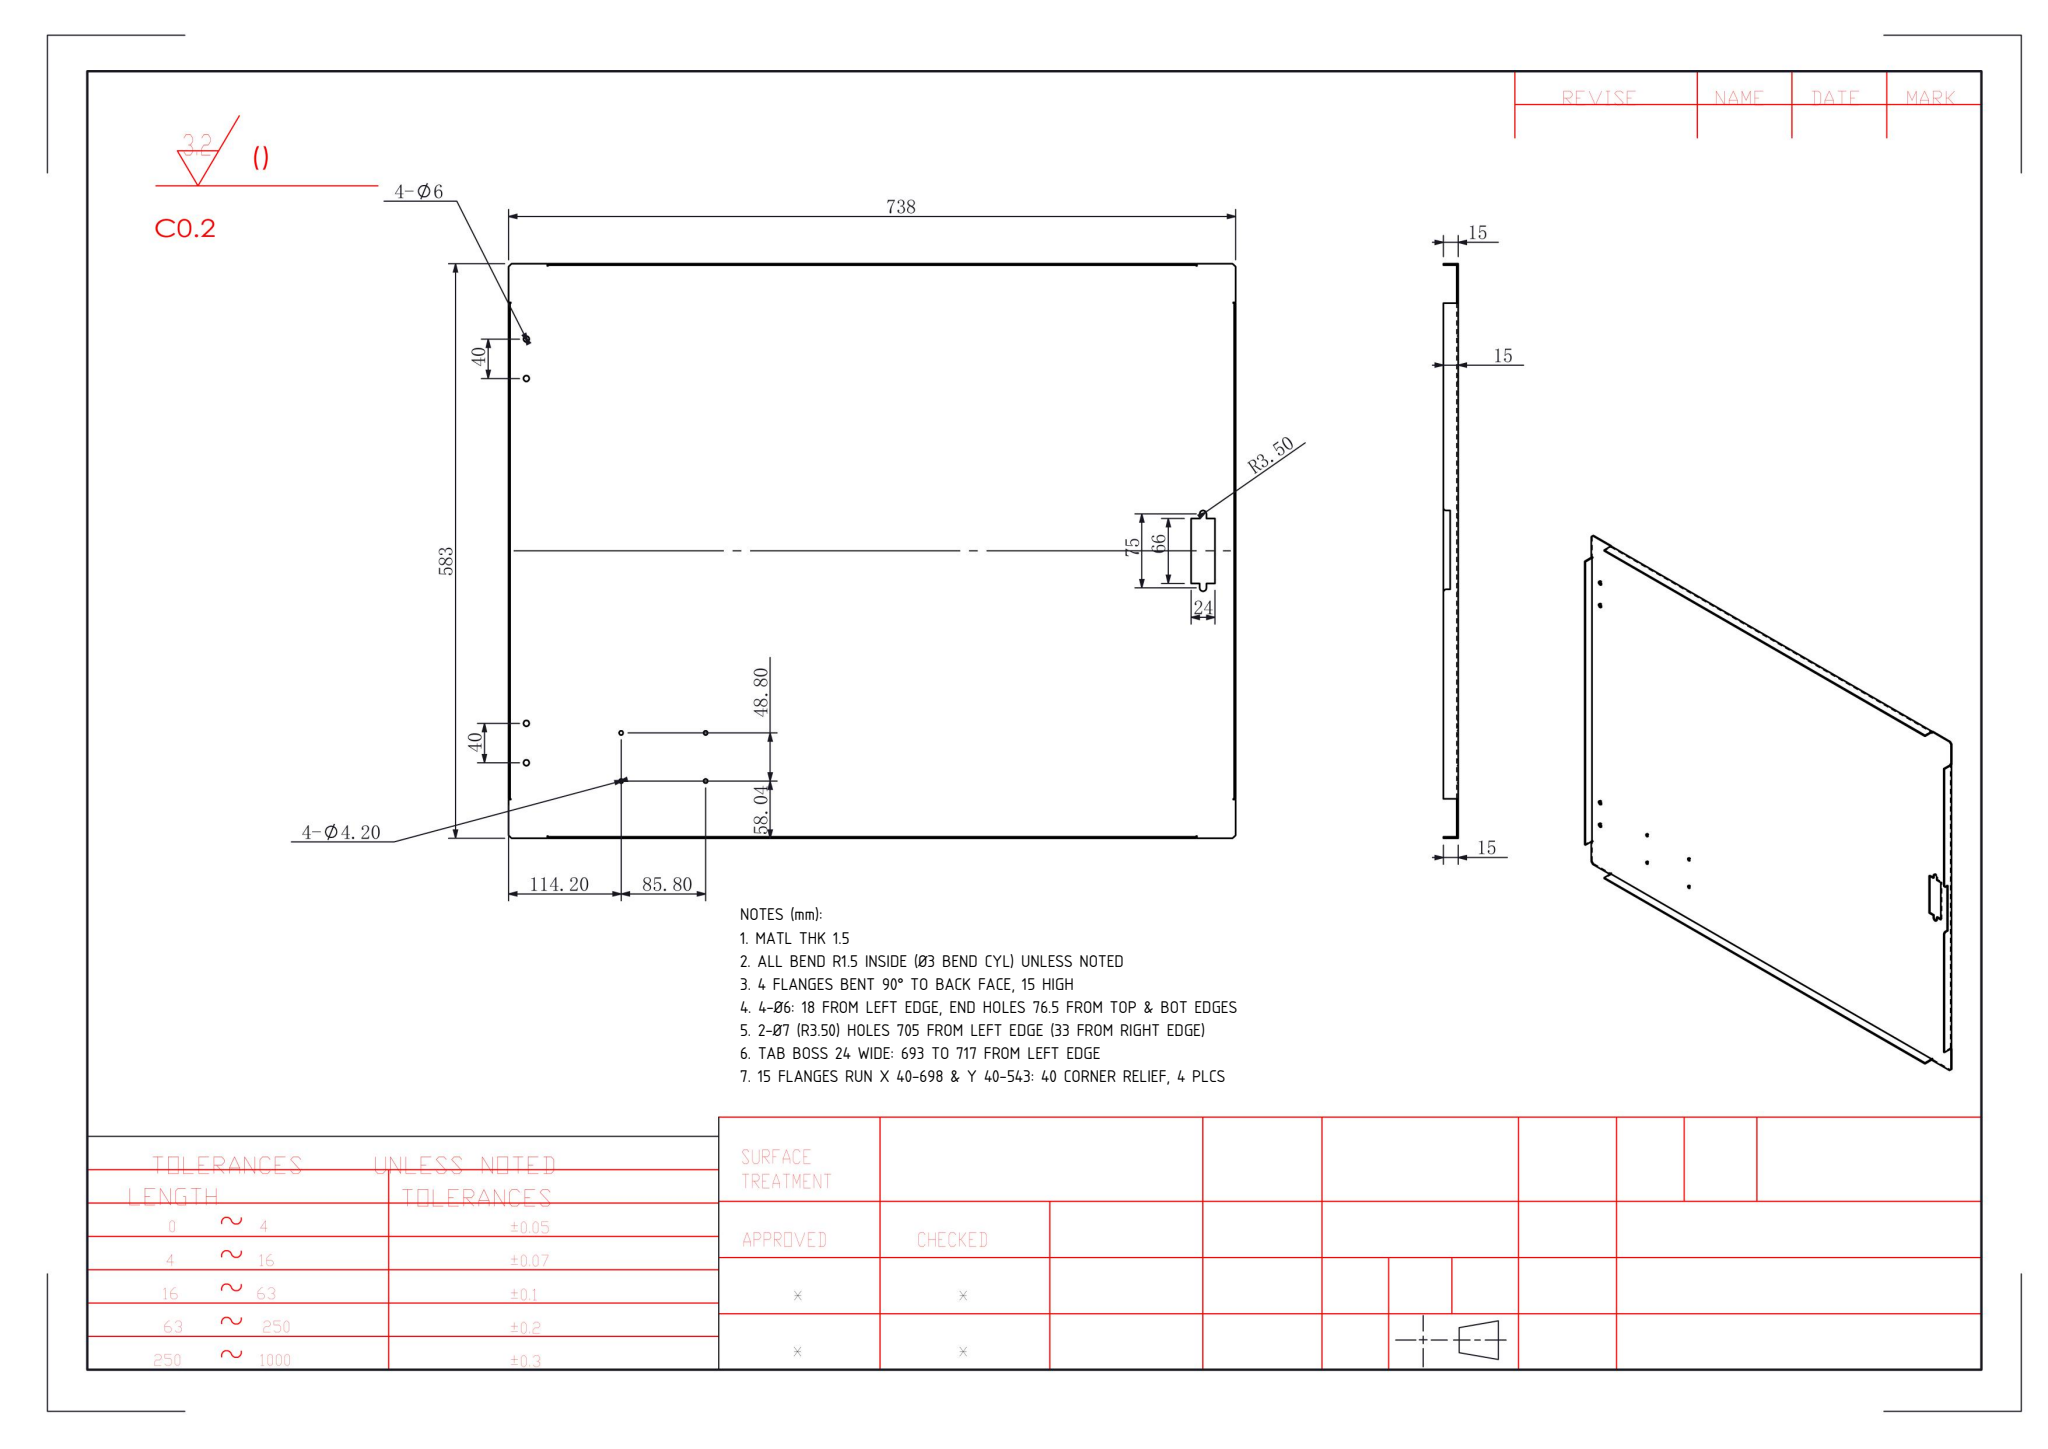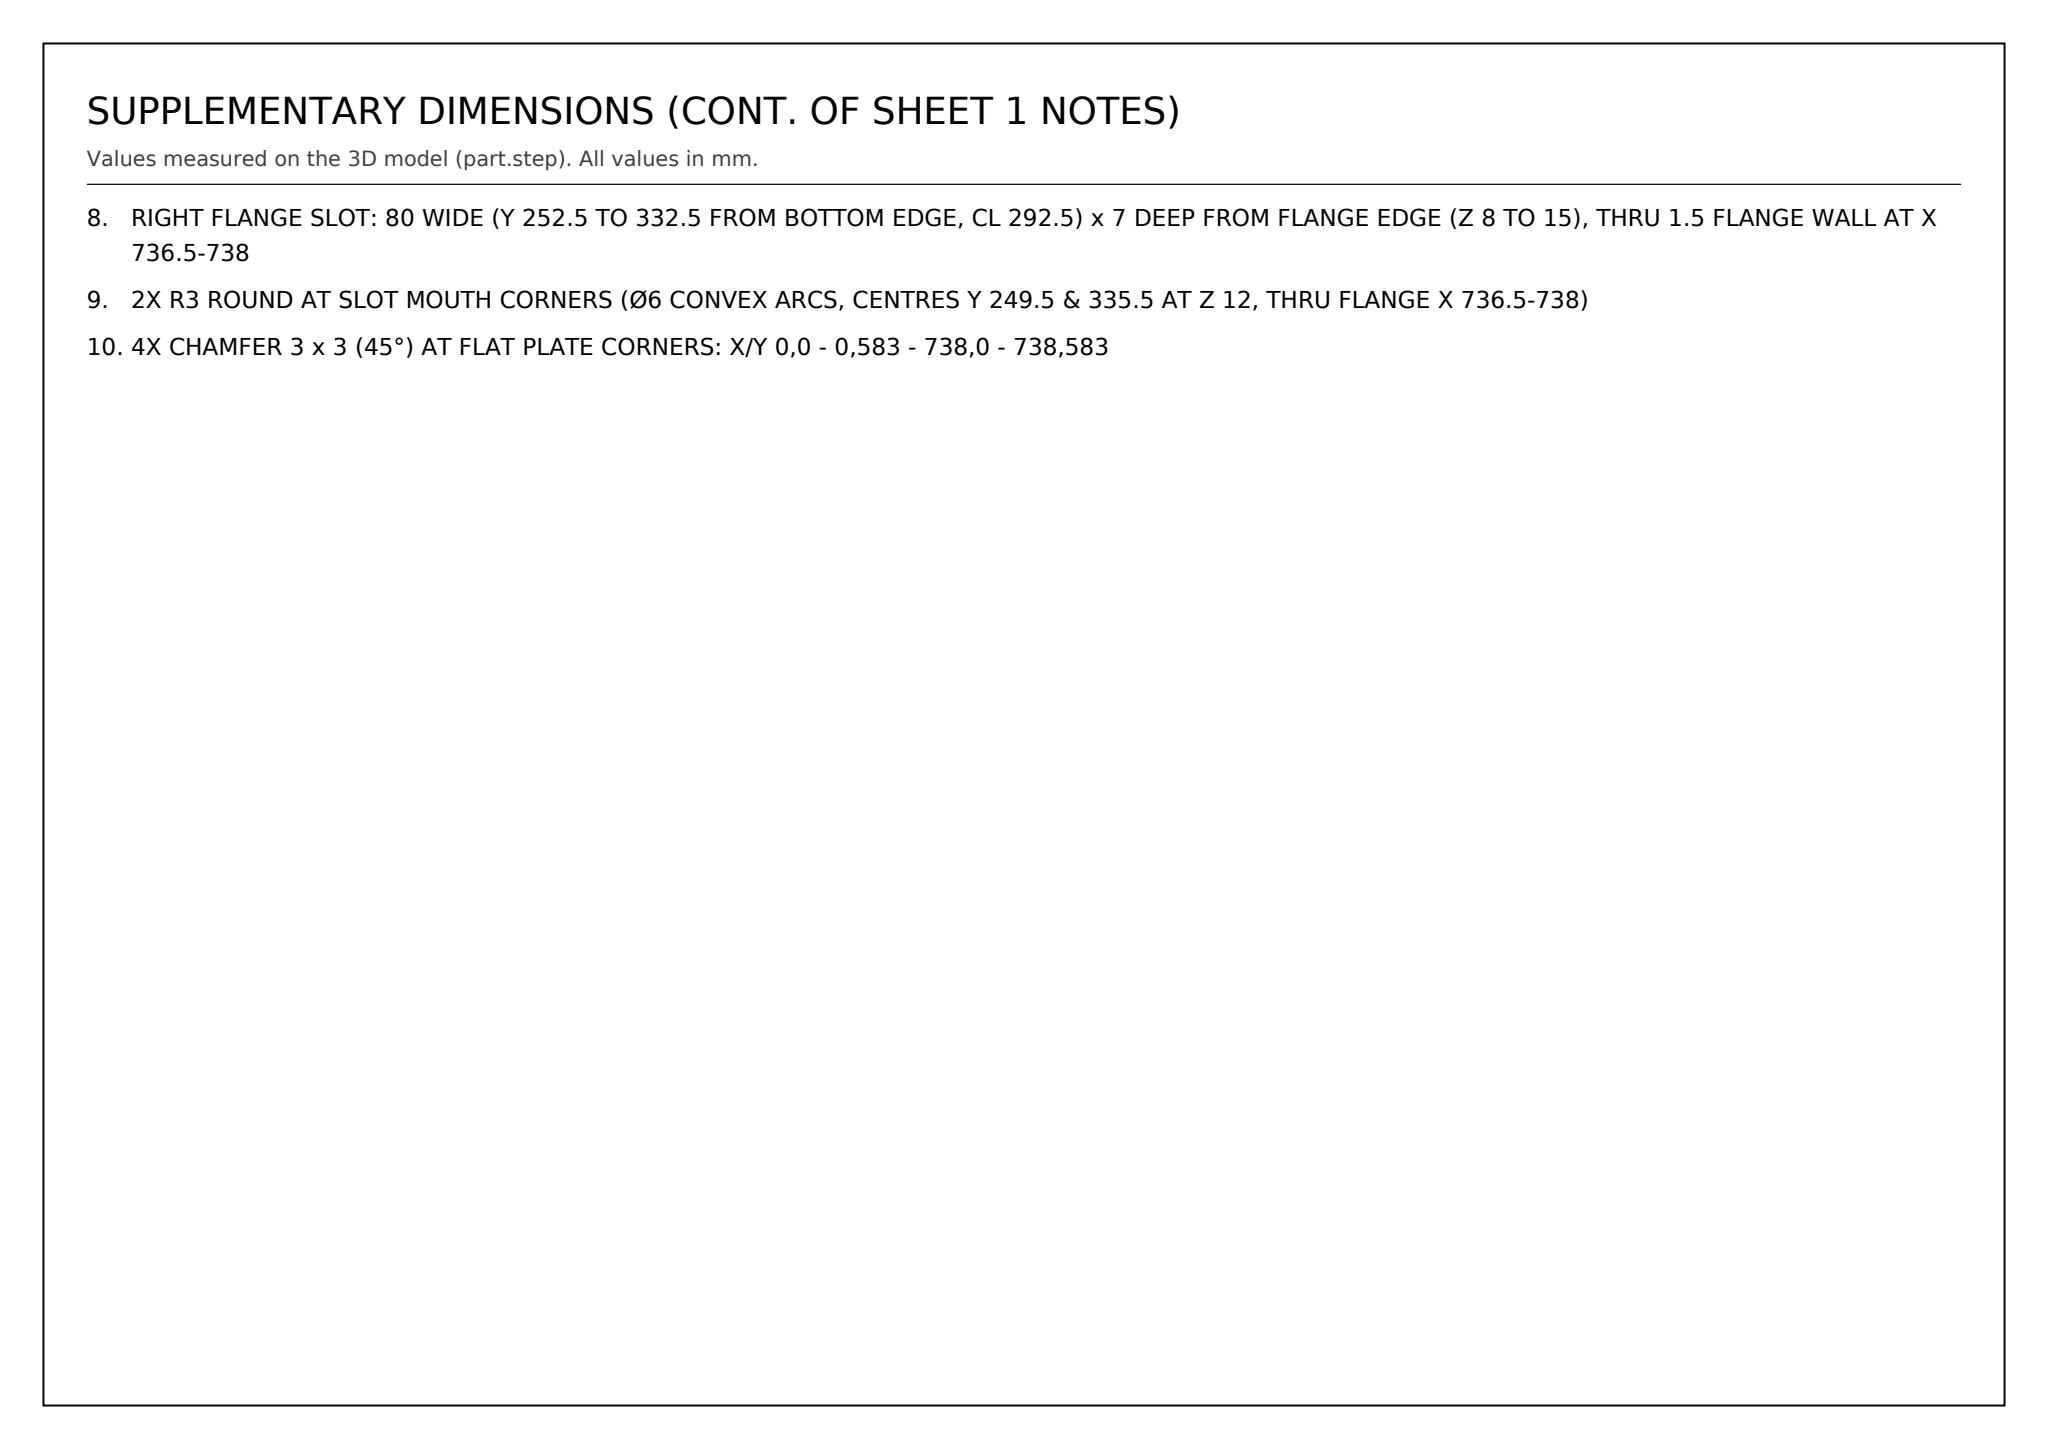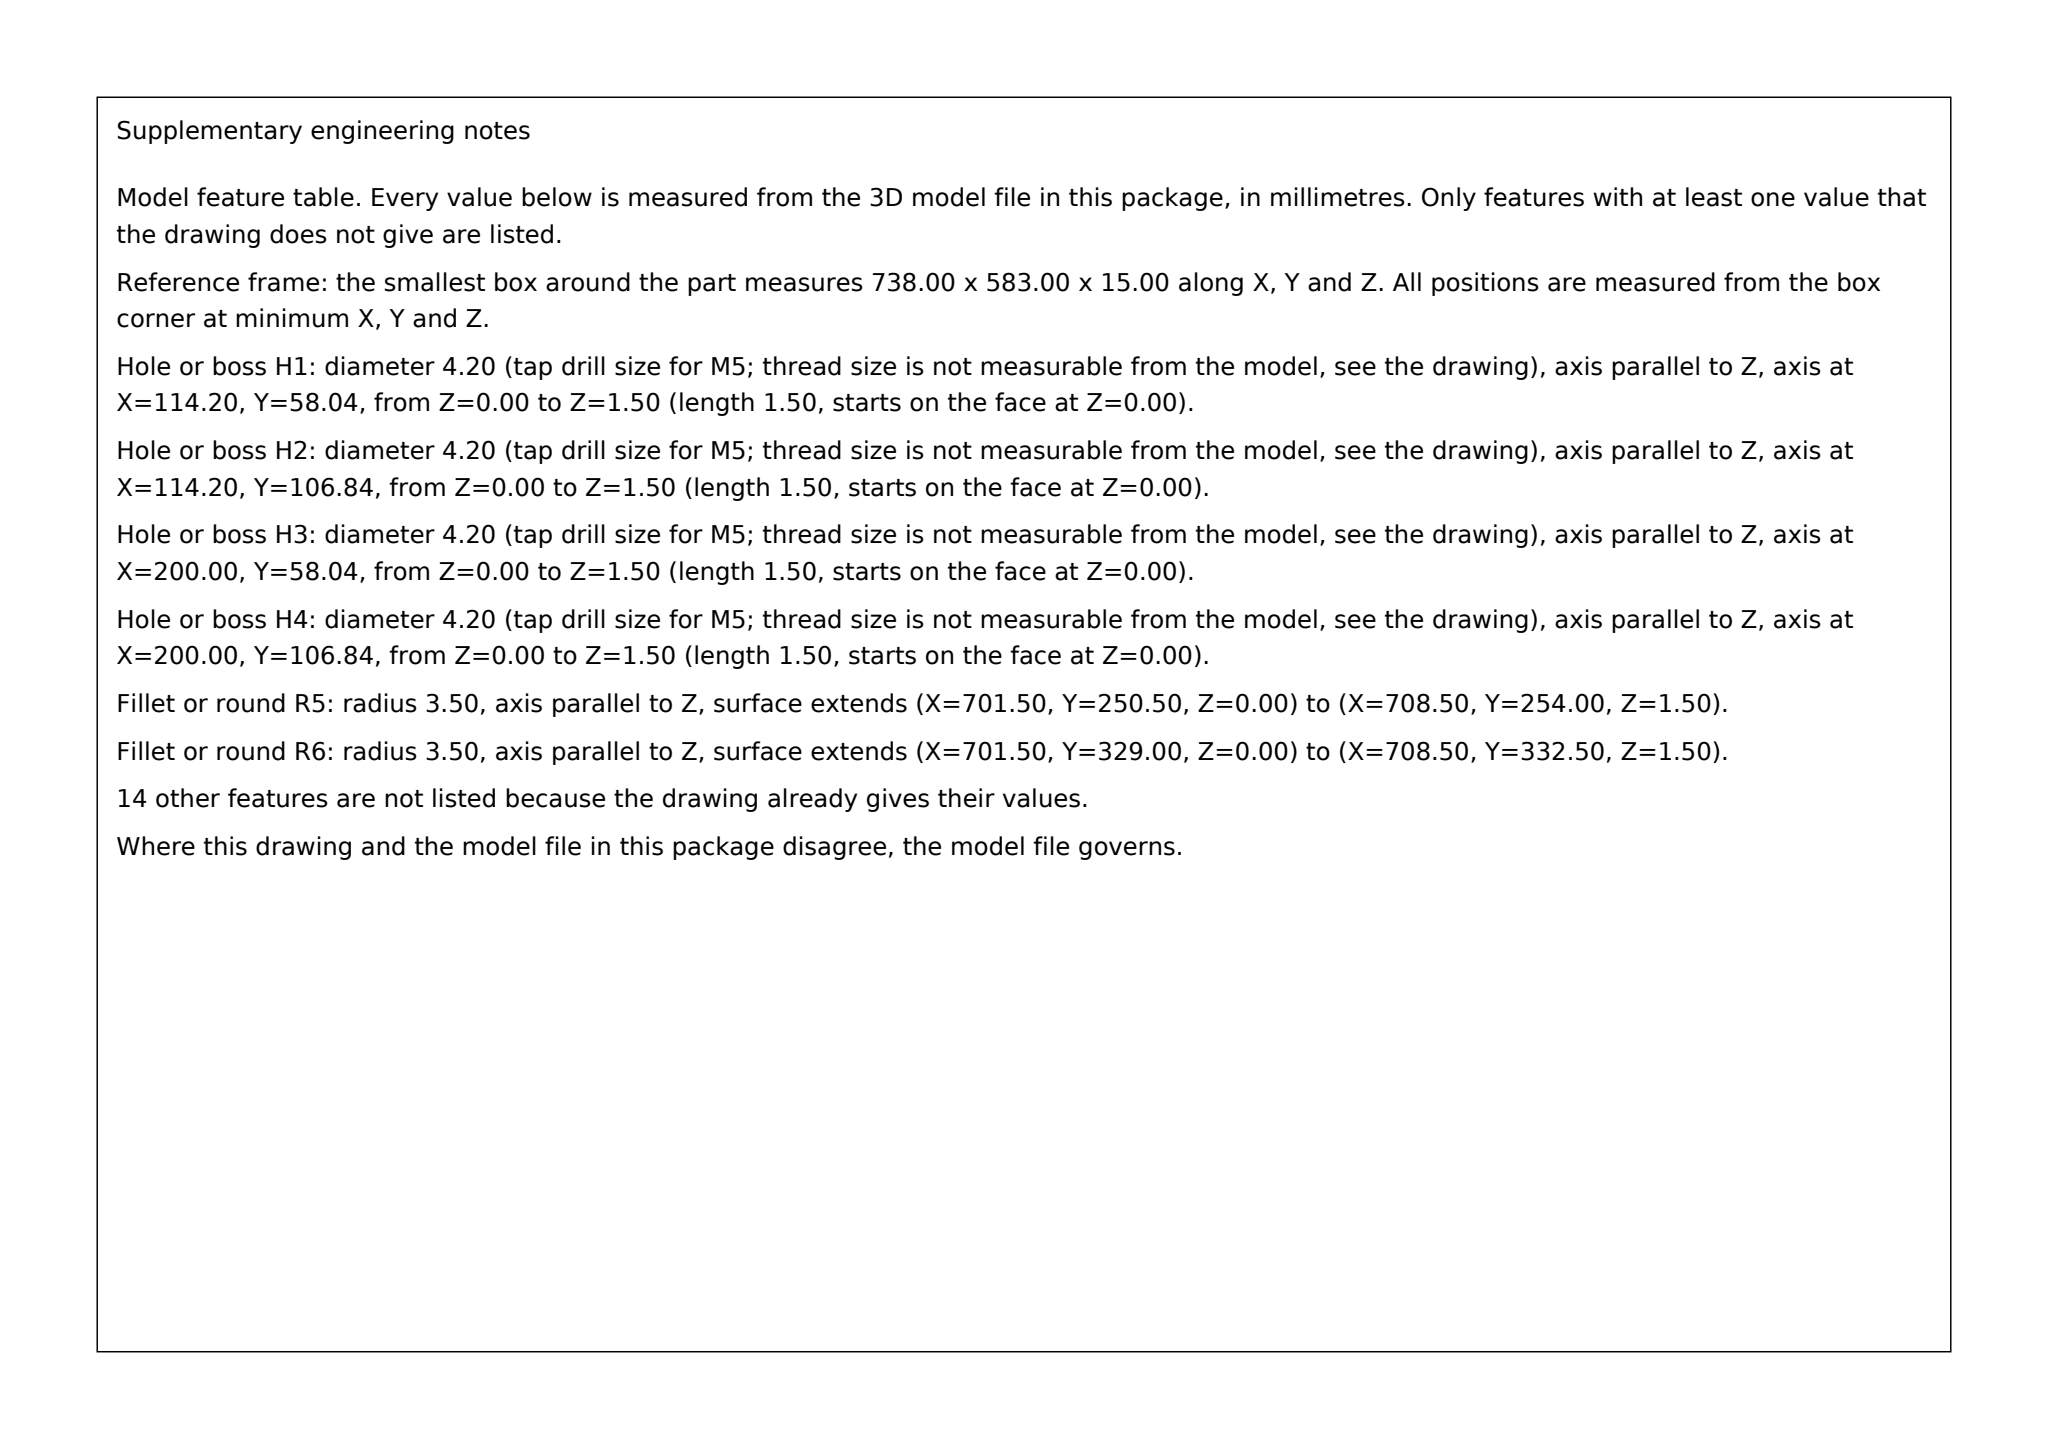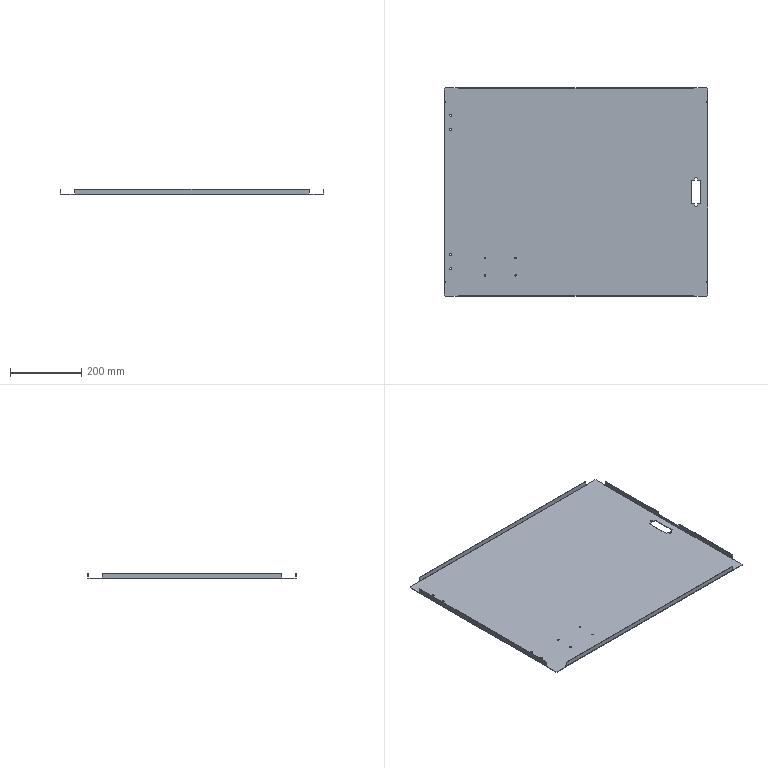Part | SolidWorks | mm | 1 solid | 104 faces | box 738 x 583 x 15 mm | volume 687606 mm3 | plane 80 | cylinder 24 | commonest cylinder face diameters 6 x10 4.2 x8 3 x4 7 x2
Drawing notes:
MATL THK 1.5 | from the solid: z planes at 0.0 and 1.5; flange walls 1.5 thk (x 0/1.5, 736.5/738)
ALL BEND R1.5 INSIDE (Ø3 BEND CYL) UNLESS NOTED | from the solid: cylinders Ø3.0 axis x at (y1.5,z1.5)&(y581.5,z1.5); axis y at (x1.5,z1.5)&(x736.5,z1.5)
4 FLANGES BENT 90° TO BACK FACE, 15 HIGH | from the solid: z planes 0 and 15; flange walls normal to x/y at 0-1.5 & 736.5-738, 0-1.5 & 581.5-583
4-Ø6: 18 FROM LEFT EDGE, END HOLES 76.5 FROM TOP & BOT EDGES | from the solid: Ø6 z-axis holes at (18,76.5),(18,116.5),(18,466.5),(18,506.5); 583-506.5=76.5
2-Ø7 (R3.50) HOLES 705 FROM LEFT EDGE (33 FROM RIGHT EDGE) | from the solid: Ø7 z-axis holes at x=705.0, y=254.0 & 329.0; bbox x=738
TAB BOSS 24 WIDE: 693 TO 717 FROM LEFT EDGE | from the solid: x planes at 693.0 and 717.0, 717-693=24
15 FLANGES RUN X 40-698 & Y 40-543: 40 CORNER RELIEF, 4 PLCS | from the solid: Planes x=40 & x=698 (6 each), y=40 & y=543 (6 each) bound 15-high flanges within 738x583 bbox; bend radii cyl len 658=698-40 and 503=543-40
RIGHT FLANGE SLOT: 80 WIDE (Y 252.5 TO 332.5 FROM BOTTOM EDGE, CL 292.5) x 7 DEEP FROM FLANGE EDGE (Z 8 TO 15), THRU 1.5 FLANGE WALL AT X 736.5-738 | from the solid: axis_planes y=252.5 and y=332.5, extent x [736.5,738] z [8,12]; flange outer face x=738, z range 1.5-15
2X R3 ROUND AT SLOT MOUTH CORNERS (Ø6 CONVEX ARCS, CENTRES Y 249.5 & 335.5 AT Z 12, THRU FLANGE X 736.5-738) | from the solid: cylinders: convex arc dia 6.0, axis x, pos [-,249.5,12.0] and [-,335.5,12.0], from 736.5 to 738.0, 90 deg
4X CHAMFER 3 x 3 (45°) AT FLAT PLATE CORNERS: X/Y 0,0 - 0,583 - 738,0 - 738,583 | from the solid: inclined_planes: 4 x 45/45/90 faces, size [3.0,3.0,1.5], bbox_from [0,0,0], [0,580,0], [735,0,0], [735,580,0]